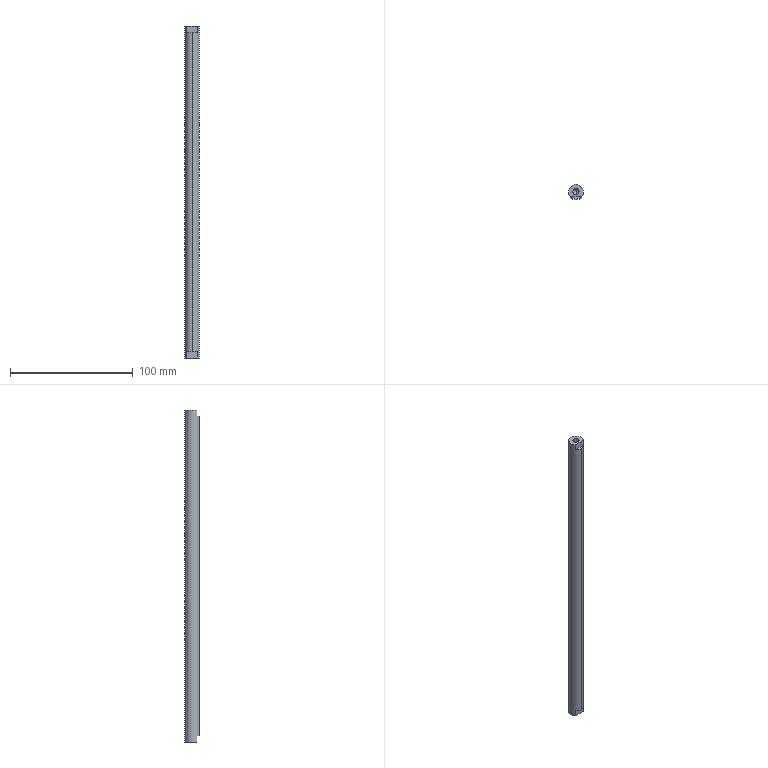CAM job | Mastercam | mm | 2 operations | part box 12 x 12 x 270
1. Contour (2D) | 10 - 10 平铣刀
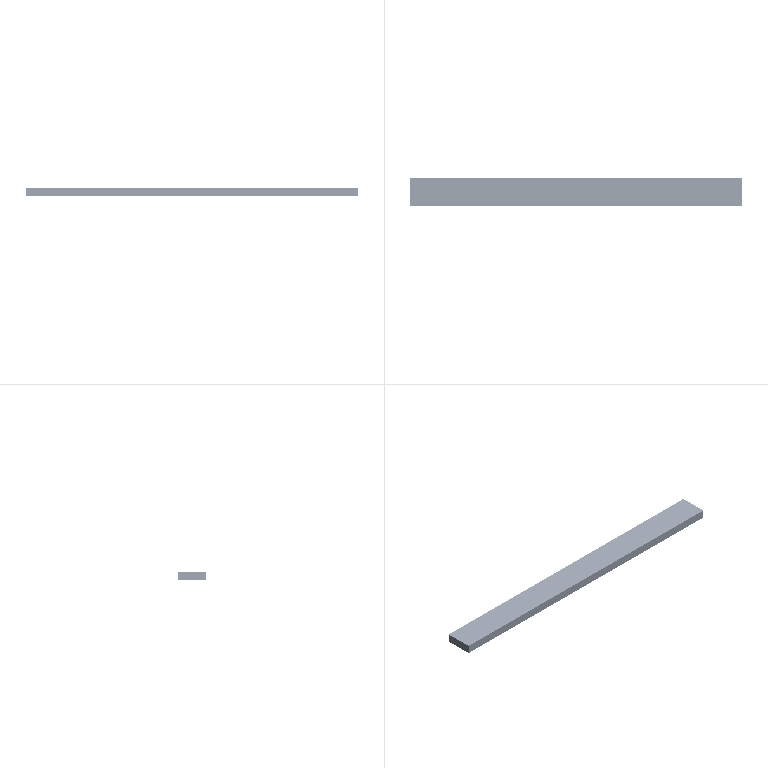2. Contour (2D) | 10 - 10 平铣刀